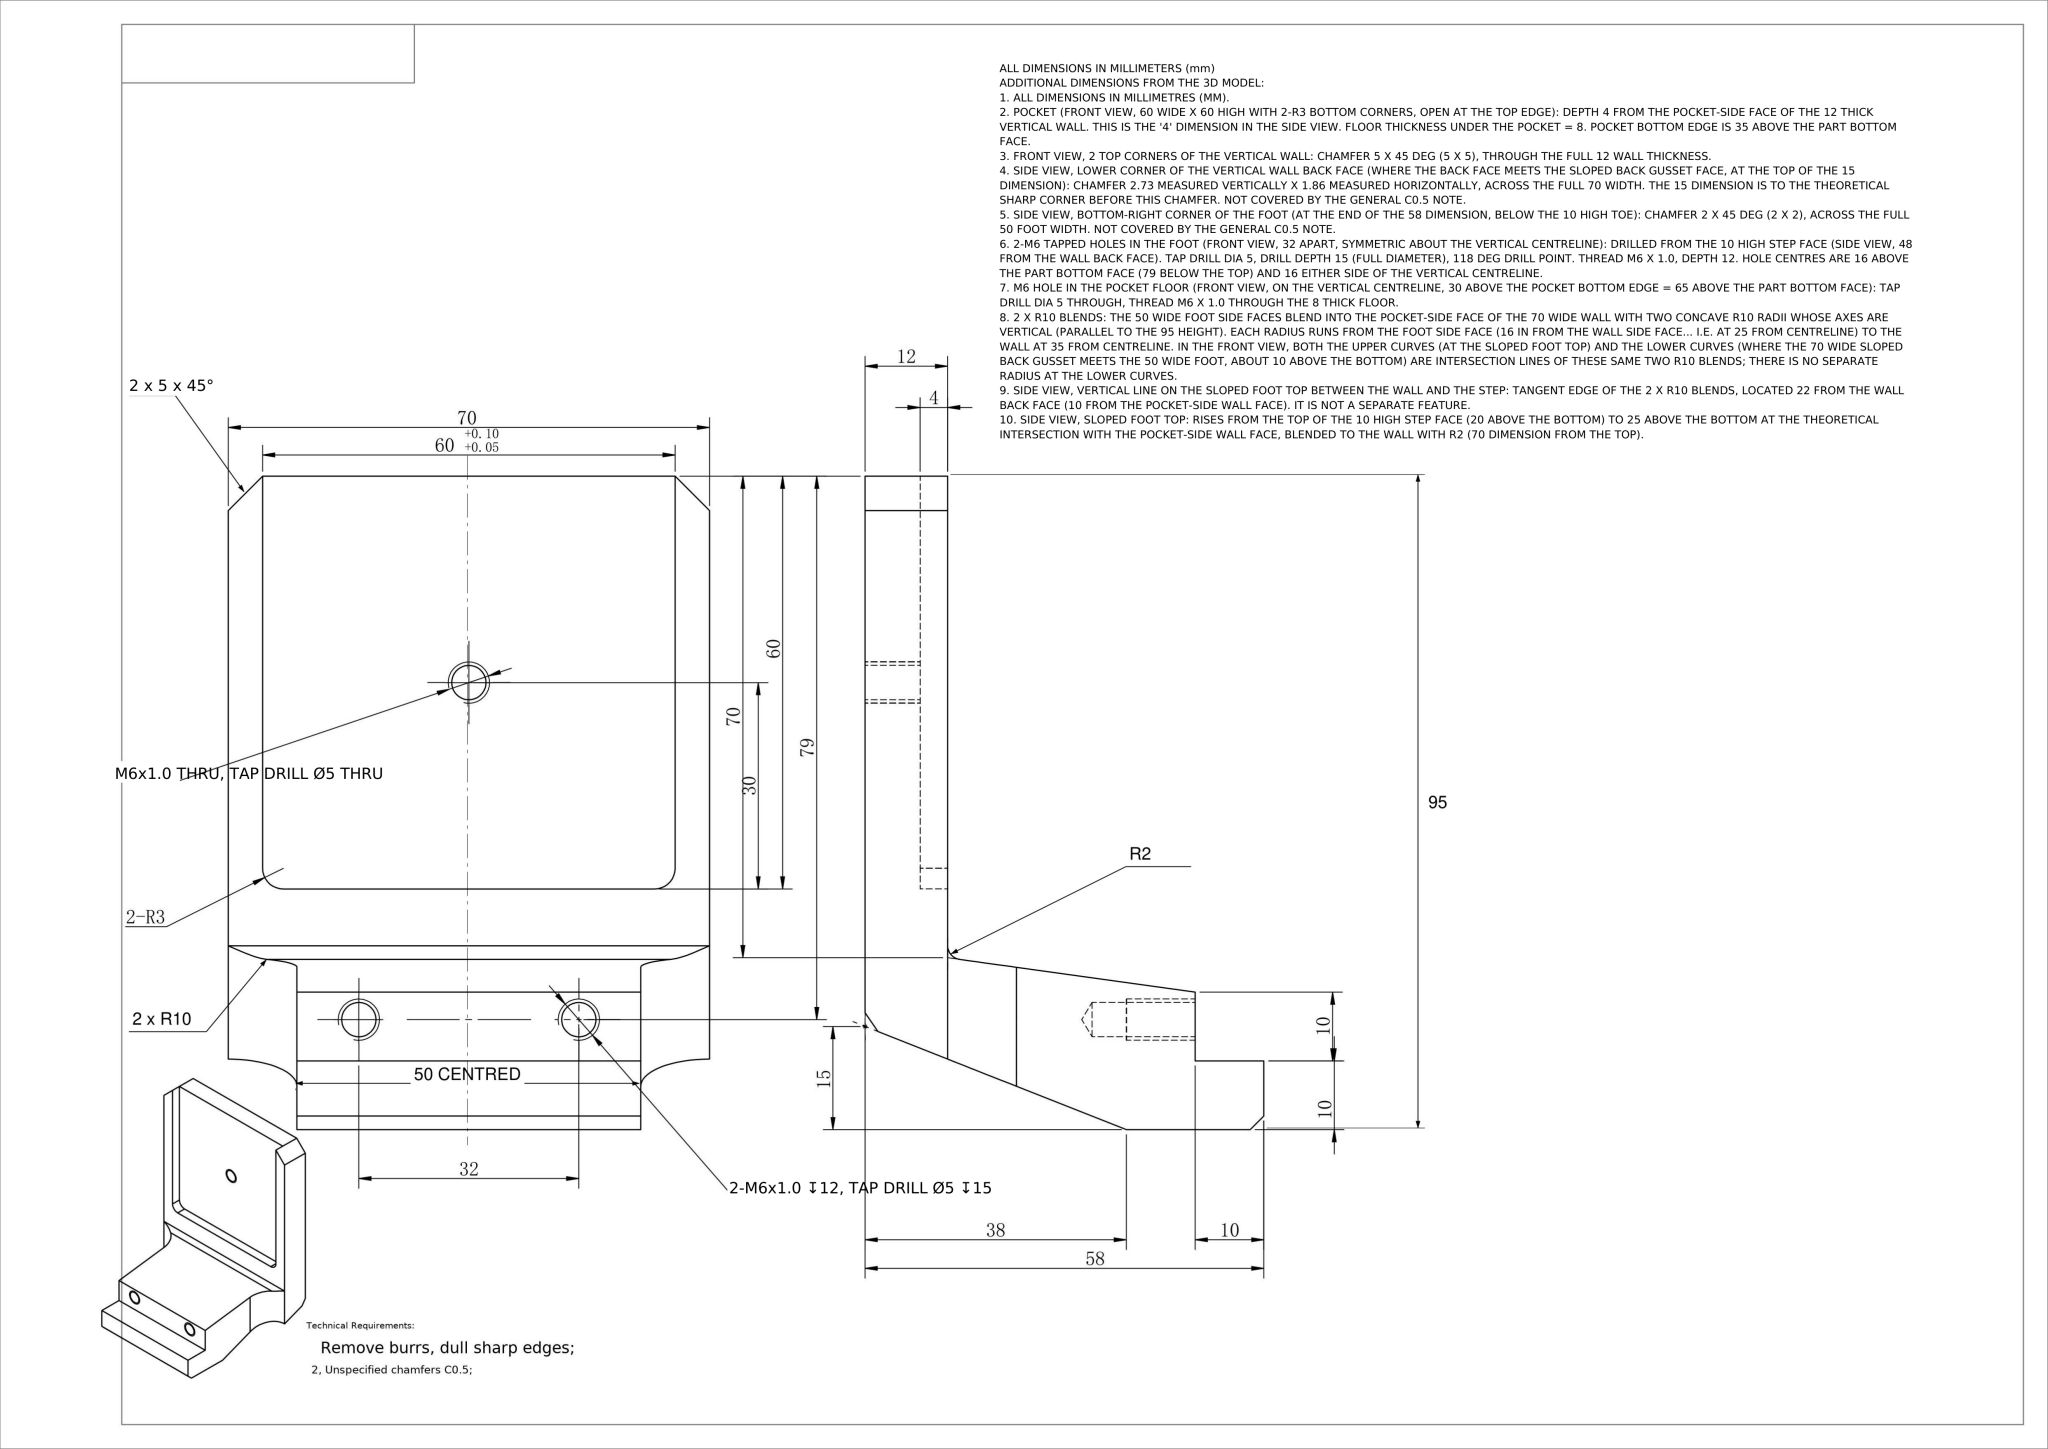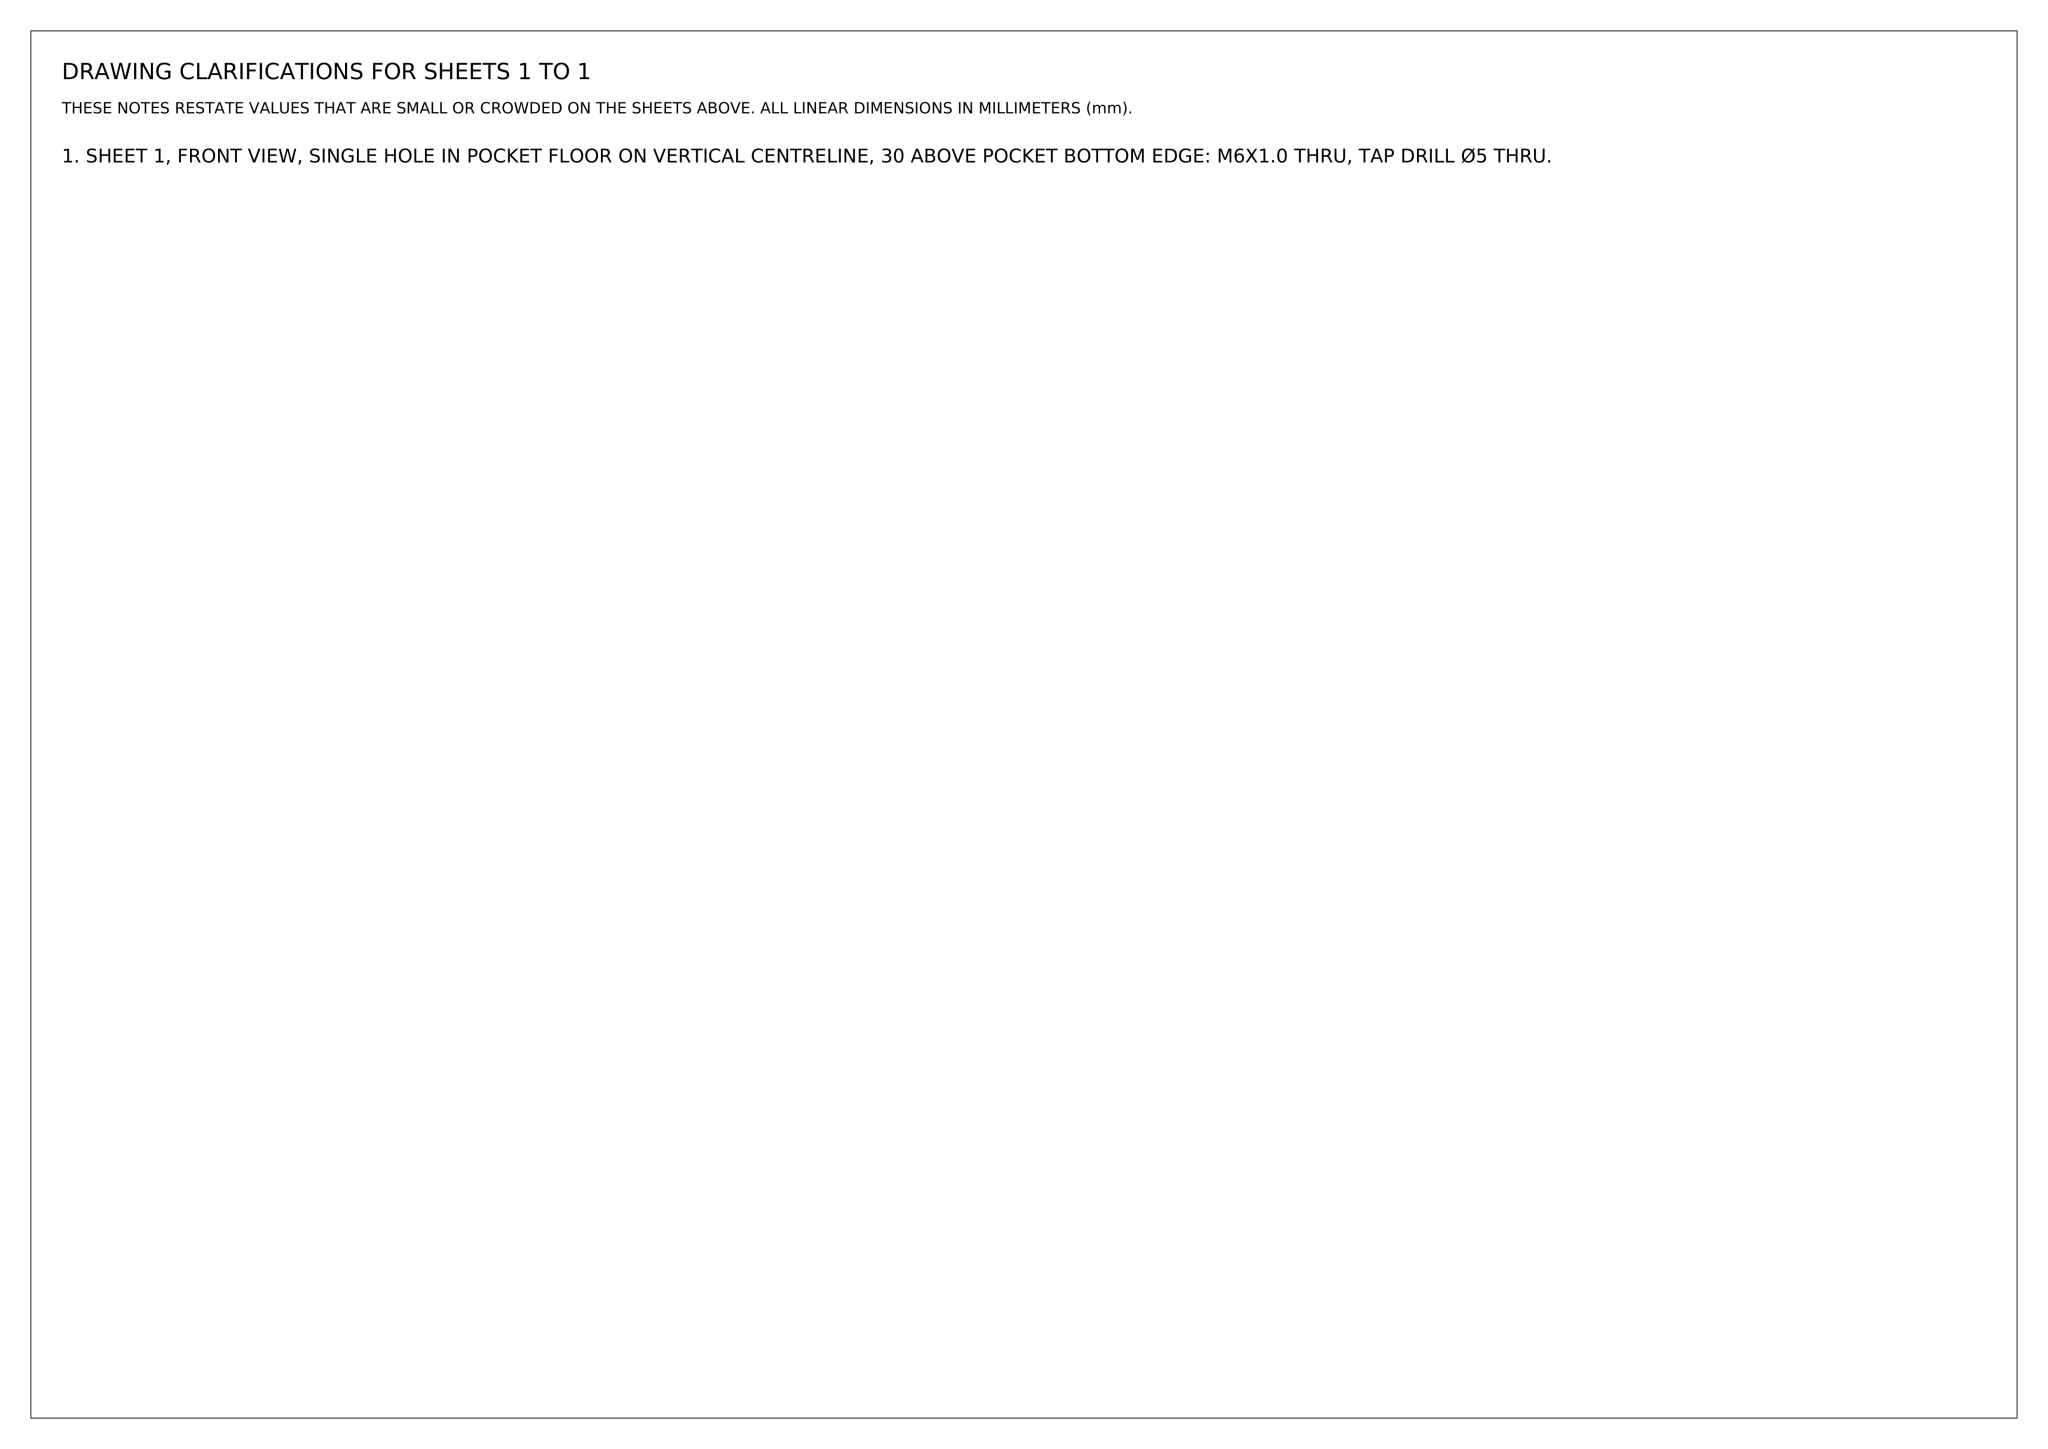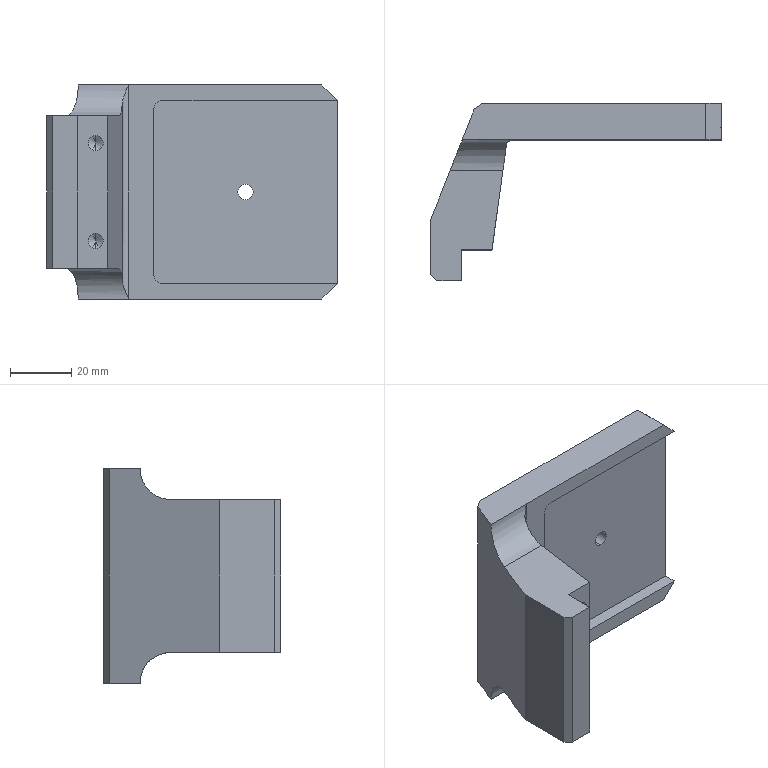Part | NX | mm | 1 solid | 36 faces | box 95 x 58 x 70 mm | volume 93035 mm3 | plane 21 | cylinder 11 | cone 4 | commonest cylinder face diameters 5 x6 6 x2 20 x2 4 x1